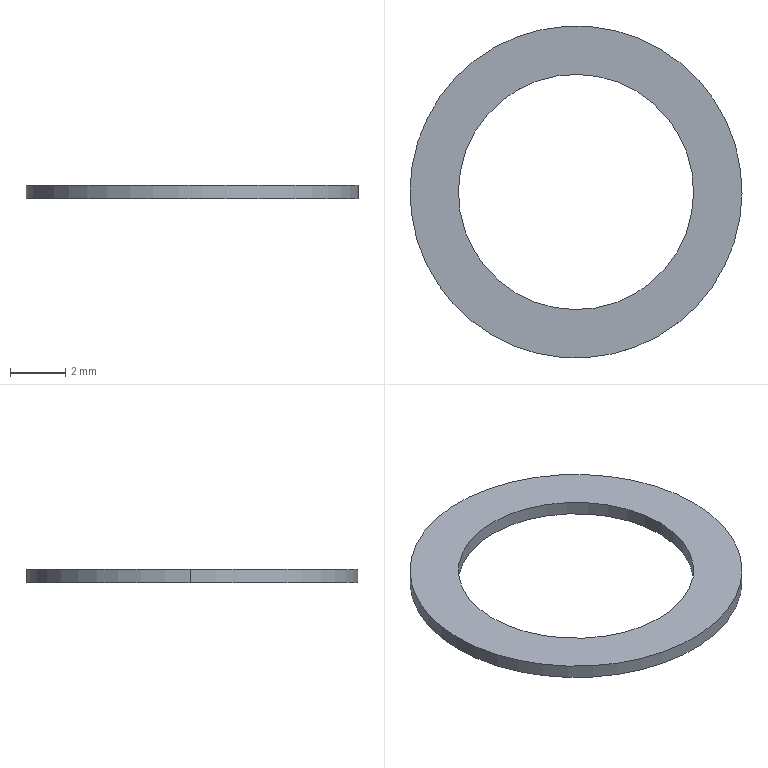Component | SolidWorks | --MA18S20041JR-SHuangGWGasket1-5 | 1 solid | 6 faces | box 12 x 12 x 0.5 mm | volume 28 mm3 | cylinder 4 | plane 2 | commonest cylinder face diameters 8.5 x2 12 x2
build123d program:
from build123d import *

# Parameters (mm, degrees)
SKETCH1_R           = 6
SKETCH1_R_2         = 4.25
BOSS_EXTRUDE1_DEPTH = 0.5


with BuildPart() as part:
    # Sketch1 → Boss-Extrude1 (new body)
    with BuildSketch(Plane.XY):
        Circle(SKETCH1_R)
        Circle(SKETCH1_R_2, mode=Mode.SUBTRACT)
    extrude(amount=BOSS_EXTRUDE1_DEPTH)


solid = part.part

# Placed as in the assembly
solid = solid.moved(Location((-165.956, 96.699, 43), (0, 0, 0)))